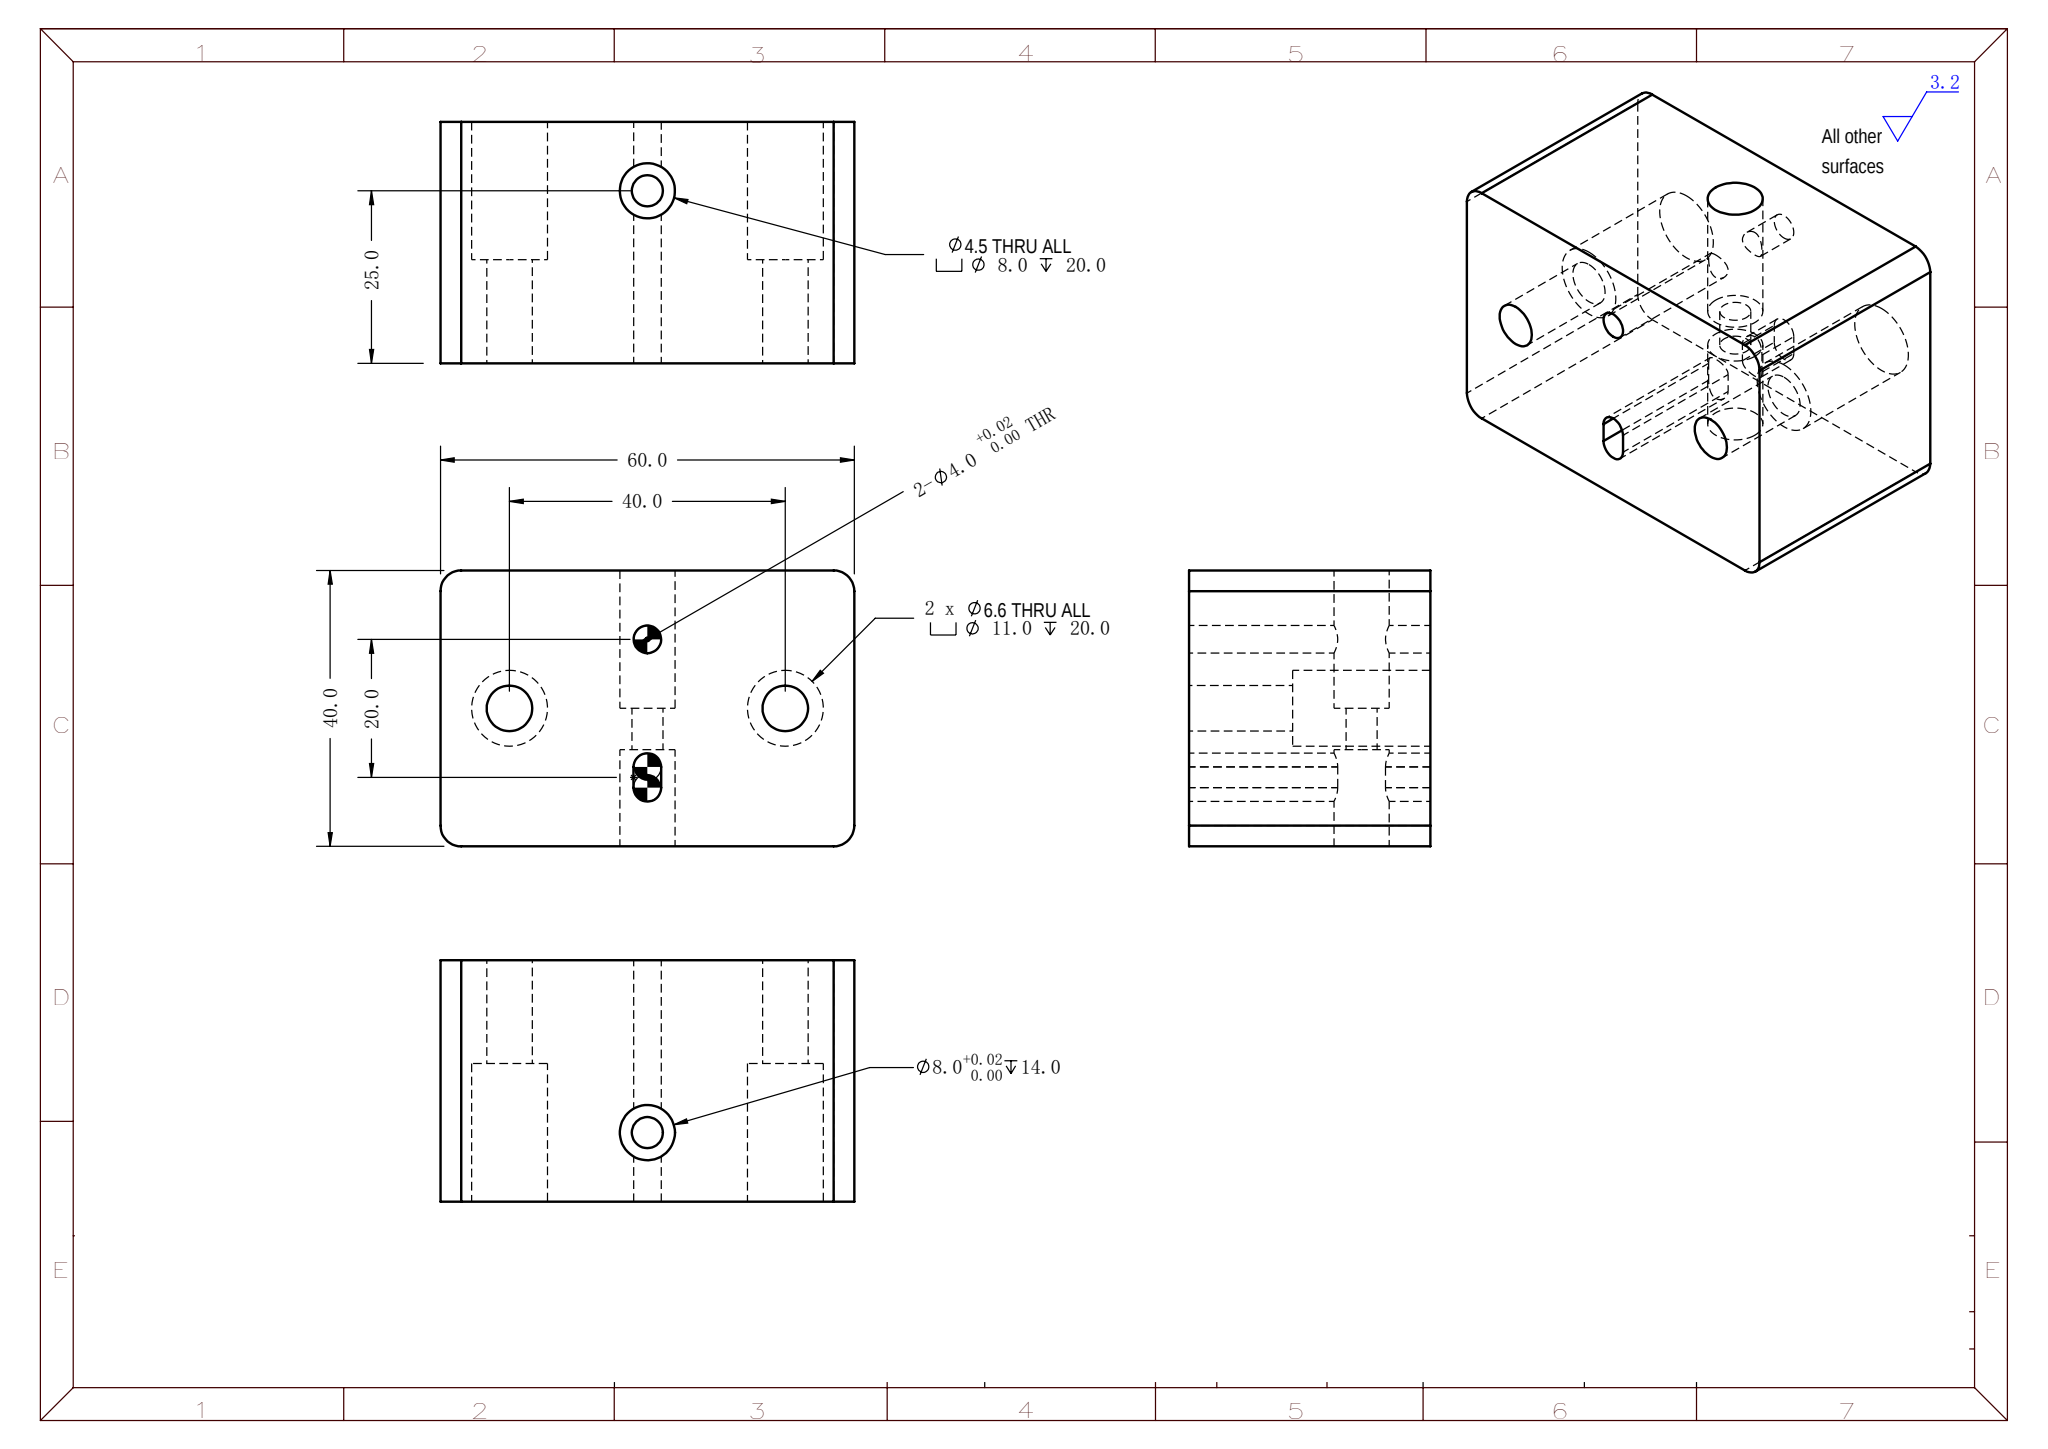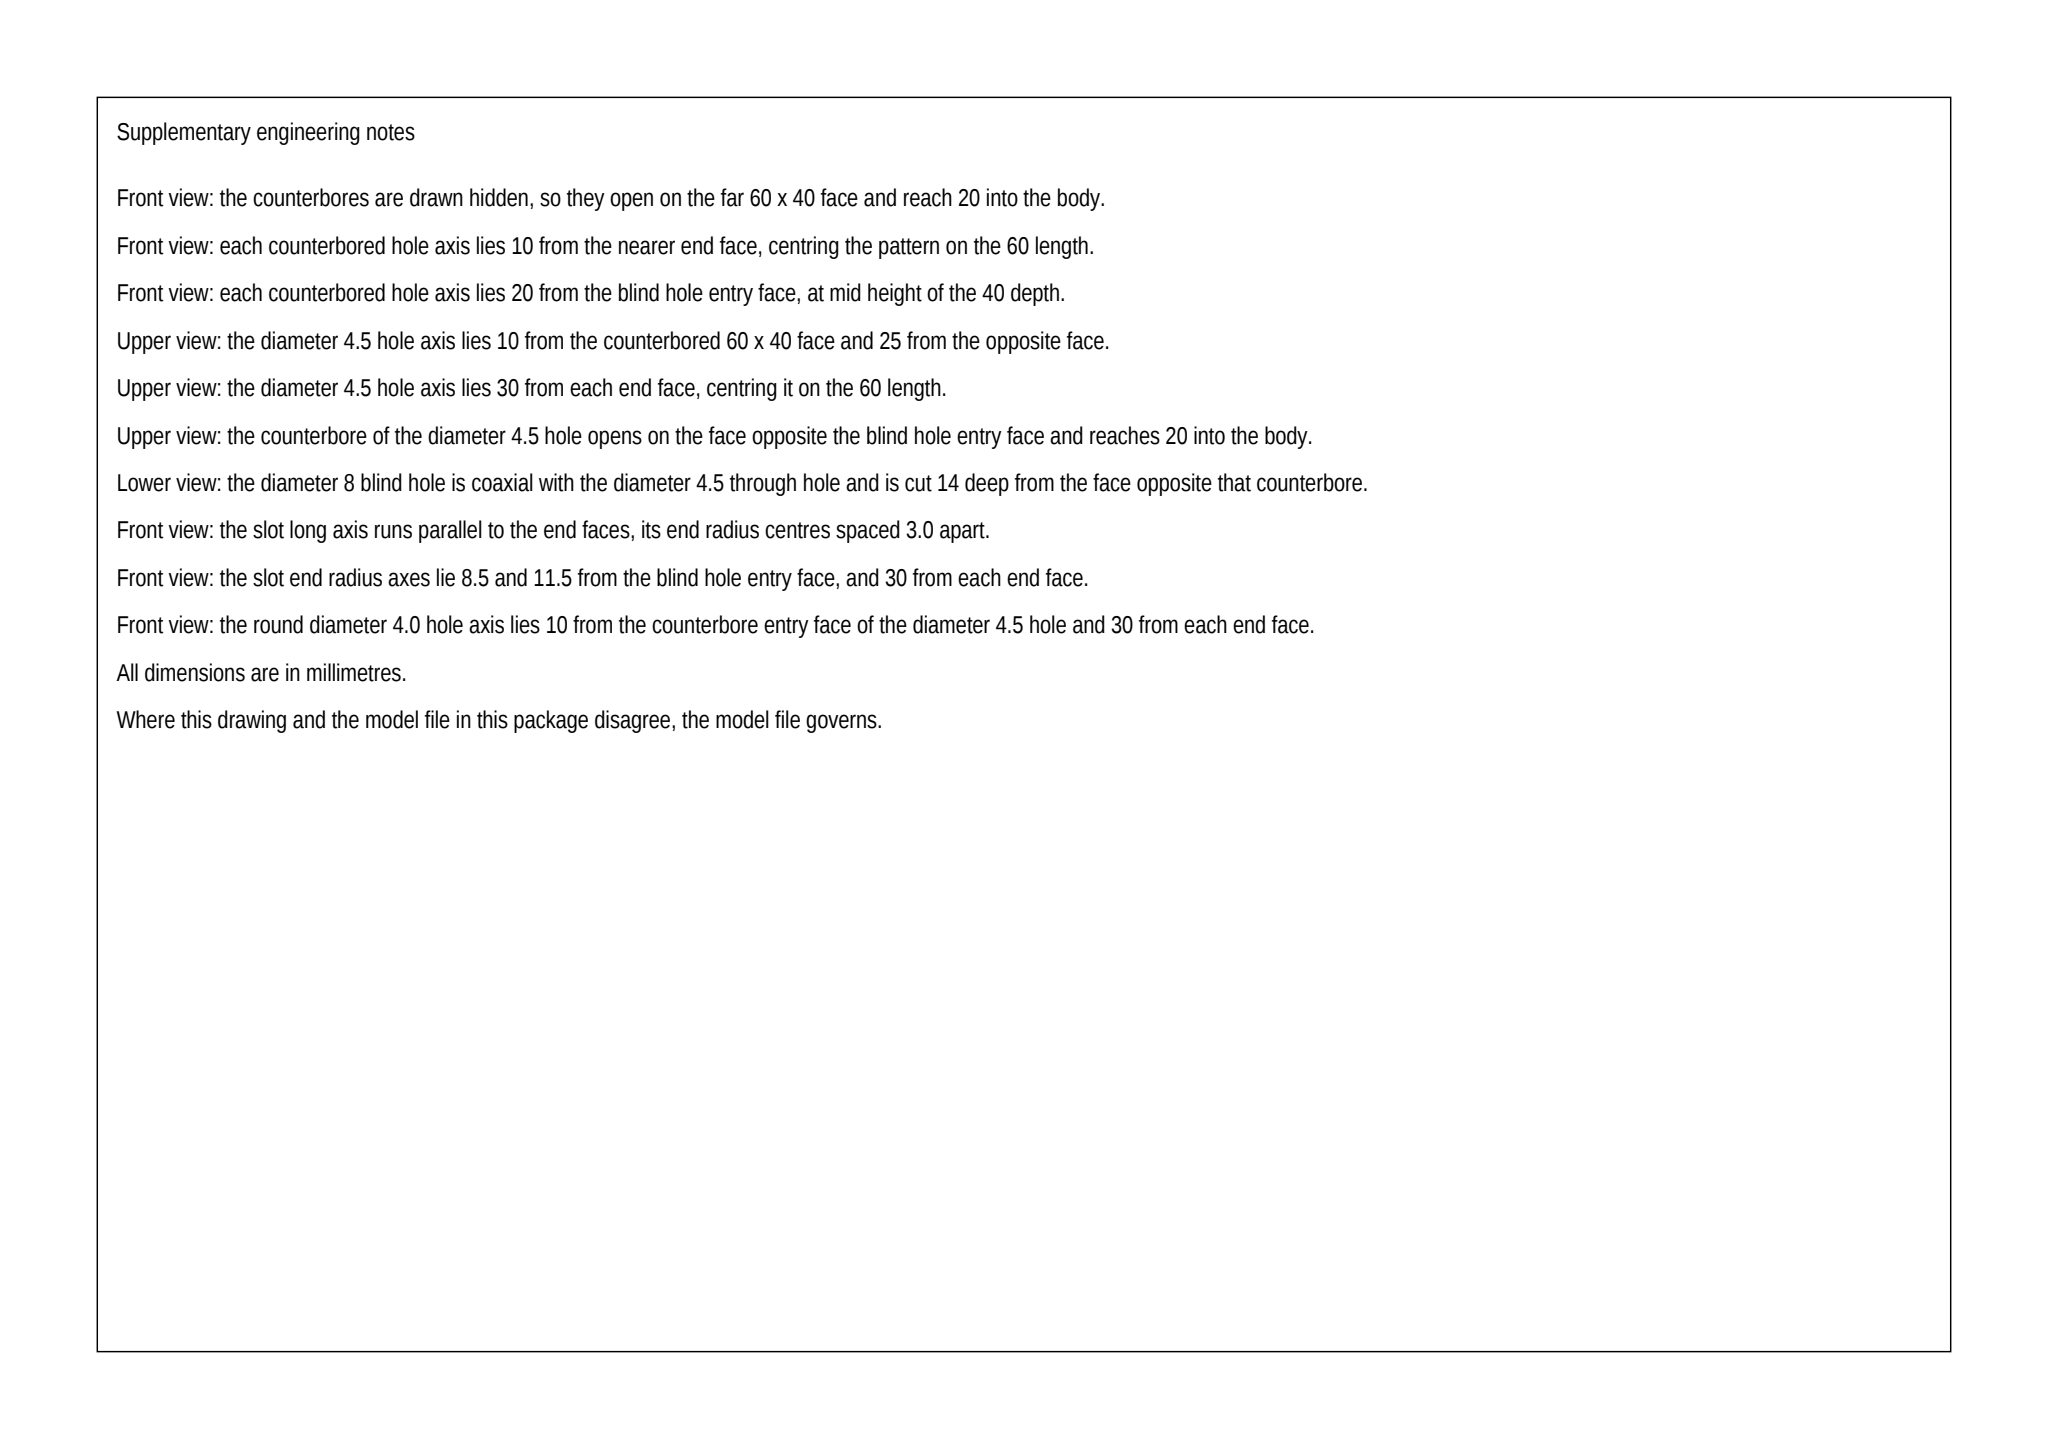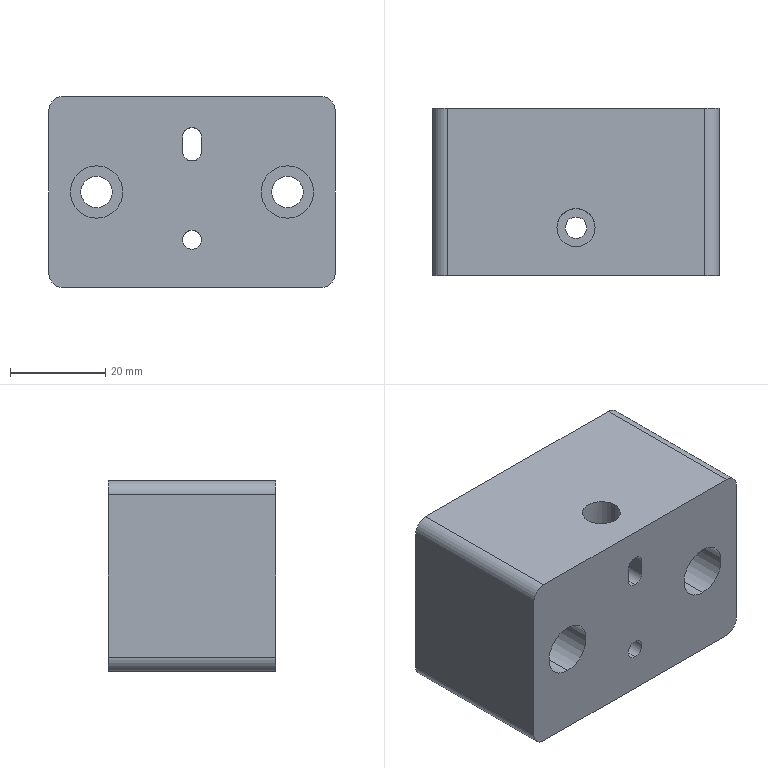Part | SolidWorks | mm | 1 solid | 42 faces | box 60 x 35 x 40 mm | volume 76084 mm3 | cylinder 28 | plane 14 | commonest cylinder face diameters 4 x10 8 x4 11 x4 6.6 x4 6 x4 4.5 x2
Drawing notes:
UPPER Ø4.0 CROSS HOLE OBROUND, 3.0 SLOT LG (Z28.5 & Z31.5) THRU | from the solid: 4.0 dia y-axis bores at z=28.5 and z=31.5, length 6.54+21.54 = THRU
4X R3.0 ON VERT CORNERS, FULL 35.0 LG (FRONT VIEW) | from the solid: convex arc dia 6.0 axis y at (3,3),(3,37),(57,3),(57,37), y 0->35
Ø4.0 +0.02/0 THRU 35.0; CL 30 FROM LH END, 10 UP FROM BOT | from the solid: hole dia 4.0 axis y at x=30,z=10, y 0->6.5 and 13.5->35 (bbox 60x35x40)
DEL DUP LEADER: 1X Ø4.0 +0.02/0 THRU, NOT 2X | from the solid: only one dia 4.0 round bore, axis y at x=30,z=10, split by Ø8 vert bore
SLOT 4.0W X 7.0LG R2 ENDS THRU 35.0, CL 30 UP, 30 FROM LH END | from the solid: concave dia 4.0 arcs at z=28.5 & 31.5, x=30, planes x=28/x=32, y 0->35
build123d program:
from build123d import *

# Parameters (mm, degrees)
SKETCH1_W                                       = 60
SKETCH1_H                                       = 40
SKETCH1_R                                       = 2
BOSS_EXTRUDE1_DEPTH                             = 17.5
FILLET1_R                                       = 3
M6_HEX_SOCKET_HEAD_CAP_SCREW_CBORE1_D           = 6.6
M6_HEX_SOCKET_HEAD_CAP_SCREW_CBORE1_CBORE_D     = 11
M6_HEX_SOCKET_HEAD_CAP_SCREW_CBORE1_CBORE_DEPTH = 20
SKETCH4_R                                       = 4
CUT_EXTRUDE1_DEPTH                              = 14
M4_HEX_SOCKET_HEAD_CAP_SCREW_CBORE1_D           = 4.5
M4_HEX_SOCKET_HEAD_CAP_SCREW_CBORE1_CBORE_D     = 8
M4_HEX_SOCKET_HEAD_CAP_SCREW_CBORE1_CBORE_DEPTH = 20


with BuildPart() as part:
    # Sketch1 → Boss-Extrude1 (new, symmetric)
    with BuildSketch(Plane(origin=(0, 0, 0), x_dir=(1, 0, 0), z_dir=(0, 1, 0))):
        Rectangle(SKETCH1_W, SKETCH1_H)
        with Locations(Location((0, 10, 0), (0, 0, 270))):
            Circle(SKETCH1_R, mode=Mode.SUBTRACT)
        with BuildLine():
            Line((-2, -11.5), (-2, -8.5))
            ThreePointArc((-2, -8.5), (0, -6.5), (2, -8.5))
            Line((2, -8.5), (2, -11.5))
            ThreePointArc((2, -11.5), (0, -13.5), (-2, -11.5))
        make_face(mode=Mode.SUBTRACT)
    extrude(amount=BOSS_EXTRUDE1_DEPTH, both=True)

    # Fillet1
    fillet1_edges = [part.edges().sort_by_distance(p)[0] for p in [
        (-30, 0, -20),
        (30, 0, -20),
        (30, 0, 20),
        (-30, 0, 20),
    ]]
    fillet(fillet1_edges, radius=FILLET1_R)

    # M6 Hex Socket Head Cap Screw CBORE1 (through all)
    with Locations(Plane.XZ.offset(17.5)):
        with Locations((20, 0), (-20, 0)):
            CounterBoreHole(M6_HEX_SOCKET_HEAD_CAP_SCREW_CBORE1_D / 2, M6_HEX_SOCKET_HEAD_CAP_SCREW_CBORE1_CBORE_D / 2, M6_HEX_SOCKET_HEAD_CAP_SCREW_CBORE1_CBORE_DEPTH)

    # Sketch4 → Cut-Extrude1 (cut)
    with BuildSketch(Plane.XY.offset(20)):
        with Locations((0, -7.5)):
            Circle(SKETCH4_R)
    extrude(amount=-CUT_EXTRUDE1_DEPTH, mode=Mode.SUBTRACT)

    # M4 Hex Socket Head Cap Screw CBORE1 (through all)
    with Locations(Plane(origin=(0, 0, -20), x_dir=(-1, 0, 0), z_dir=(0, 0, -1))):
        with Locations((0, -7.5)):
            CounterBoreHole(M4_HEX_SOCKET_HEAD_CAP_SCREW_CBORE1_D / 2, M4_HEX_SOCKET_HEAD_CAP_SCREW_CBORE1_CBORE_D / 2, M4_HEX_SOCKET_HEAD_CAP_SCREW_CBORE1_CBORE_DEPTH)


solid = part.part